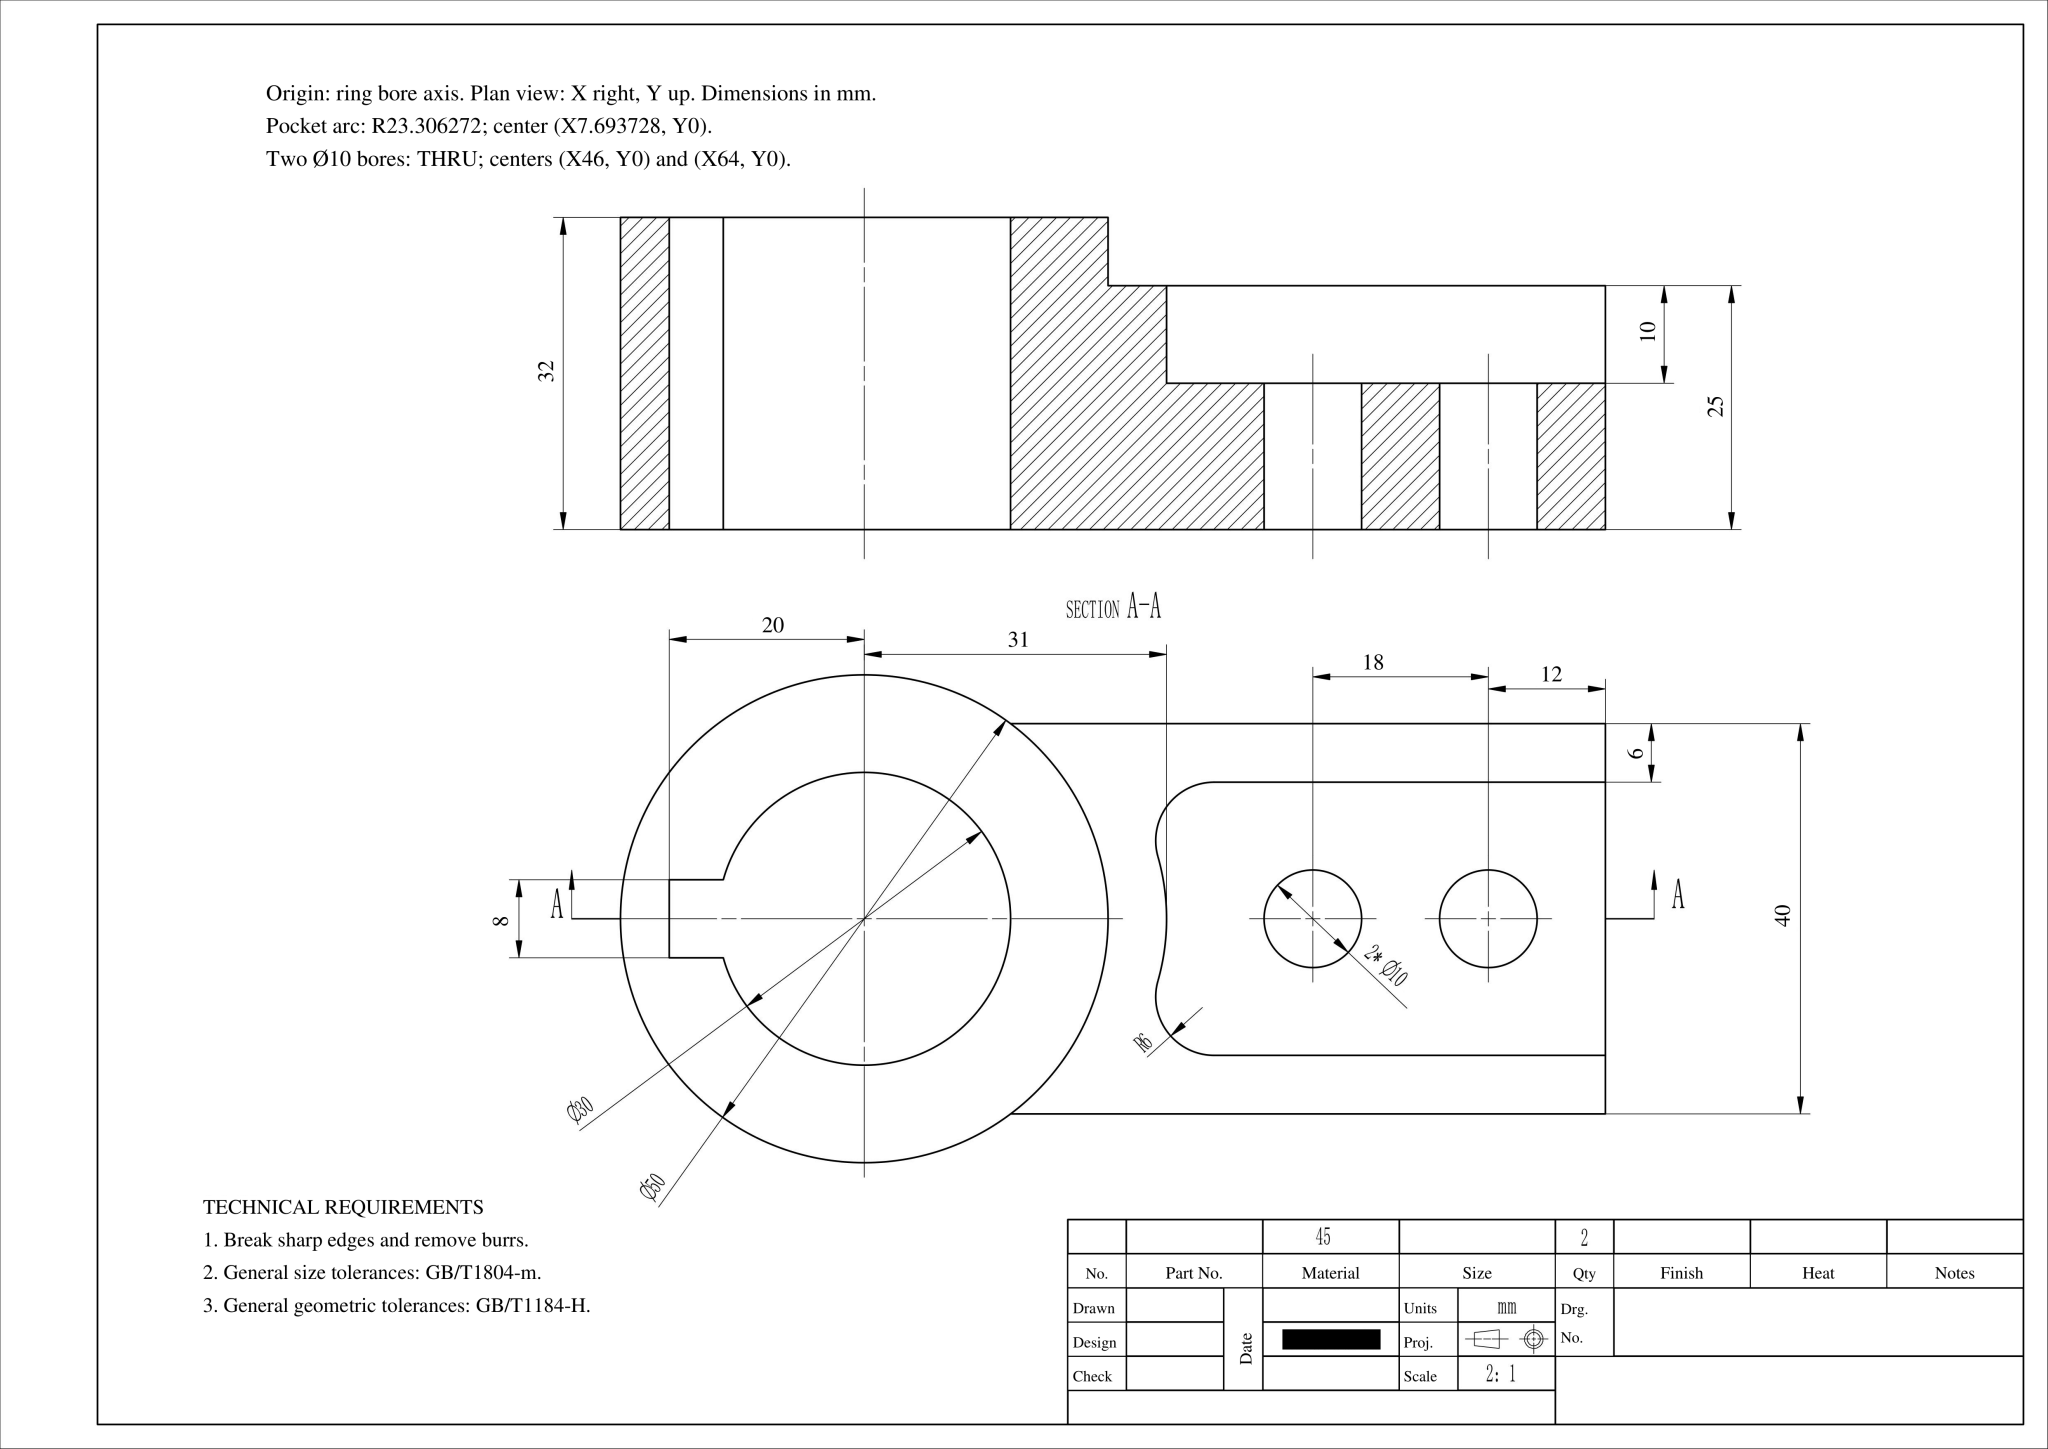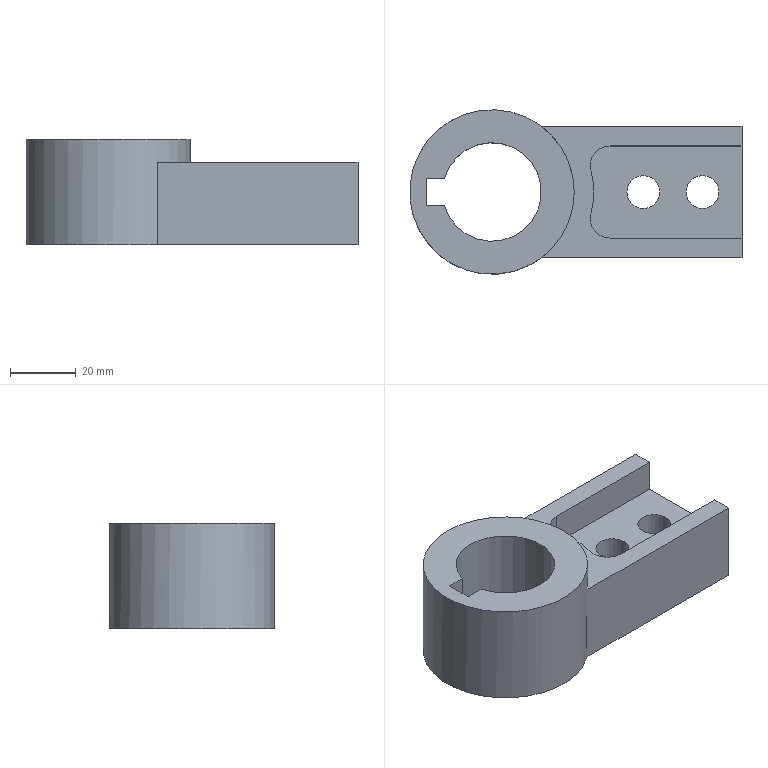Part | NX | mm | 1 solid | 19 faces | box 101 x 50 x 32 mm | volume 77891 mm3 | plane 12 | cylinder 7 | commonest cylinder face diameters 12 x2 10 x2 46.613 x1 50 x1 30 x1
STEP:
#1=CARTESIAN_POINT('',(0.,0.,0.));
#2=DIRECTION('',(0.,0.,1.));
#3=DIRECTION('',(1.,0.,0.));
#4=AXIS2_PLACEMENT_3D('',#1,#2,#3);
#5=(LENGTH_UNIT()NAMED_UNIT(*)SI_UNIT(.MILLI.,.METRE.));
#6=UNCERTAINTY_MEASURE_WITH_UNIT(LENGTH_MEASURE(0.00002),#5,'','');
#7=(NAMED_UNIT(*)PLANE_ANGLE_UNIT()SI_UNIT($,.RADIAN.));
#8=PLANE_ANGLE_MEASURE_WITH_UNIT(PLANE_ANGLE_MEASURE(0.01745),#7);
#9=DIMENSIONAL_EXPONENTS(0.,0.,0.,0.,0.,0.,0.);
#10=(CONVERSION_BASED_UNIT('',#8)NAMED_UNIT(#9)PLANE_ANGLE_UNIT());
#11=(NAMED_UNIT(*)SI_UNIT($,.STERADIAN.)SOLID_ANGLE_UNIT());
#12=(GEOMETRIC_REPRESENTATION_CONTEXT(3)GLOBAL_UNCERTAINTY_ASSIGNED_CONTEXT((#6))GLOBAL_UNIT_ASSIGNED_CONTEXT((#5,#10,#11))REPRESENTATION_CONTEXT('',''));
#13=SHAPE_REPRESENTATION('',(#4),#12);
#14=CARTESIAN_POINT('',(35.887,-14.,15.));
#15=VERTEX_POINT('',#14);
#16=CARTESIAN_POINT('',(76.,-14.,15.));
#17=VERTEX_POINT('',#16);
#18=CARTESIAN_POINT('',(35.887,-14.,15.));
#19=DIRECTION('',(1.,0.,0.));
#20=VECTOR('',#19,1.);
#21=LINE('',#18,#20);
#22=EDGE_CURVE('',#15,#17,#21,.T.);
#23=ORIENTED_EDGE('',*,*,#22,.F.);
#24=CARTESIAN_POINT('',(35.887,-14.,25.));
#25=VERTEX_POINT('',#24);
#26=CARTESIAN_POINT('',(35.887,-14.,25.));
#27=DIRECTION('',(0.,0.,-1.));
#28=VECTOR('',#27,1.);
#29=LINE('',#26,#28);
#30=EDGE_CURVE('',#25,#15,#29,.T.);
#31=ORIENTED_EDGE('',*,*,#30,.F.);
#32=CARTESIAN_POINT('',(76.,-14.,25.));
#33=VERTEX_POINT('',#32);
#34=CARTESIAN_POINT('',(76.,-14.,25.));
#35=DIRECTION('',(-1.,0.,0.));
#36=VECTOR('',#35,1.);
#37=LINE('',#34,#36);
#38=EDGE_CURVE('',#33,#25,#37,.T.);
#39=ORIENTED_EDGE('',*,*,#38,.F.);
#40=CARTESIAN_POINT('',(76.,-14.,25.));
#41=DIRECTION('',(0.,0.,-1.));
#42=VECTOR('',#41,1.);
#43=LINE('',#40,#42);
#44=EDGE_CURVE('',#33,#17,#43,.T.);
#45=ORIENTED_EDGE('',*,*,#44,.T.);
#46=EDGE_LOOP('',(#23,#31,#39,#45));
#47=FACE_OUTER_BOUND('',#46,.T.);
#48=CARTESIAN_POINT('',(76.,-14.,25.));
#49=DIRECTION('',(0.,-1.,0.));
#50=DIRECTION('',(0.,0.,-1.));
#51=AXIS2_PLACEMENT_3D('',#48,#49,#50);
#52=PLANE('',#51);
#53=ADVANCED_FACE('',(#47),#52,.F.);
#54=CARTESIAN_POINT('',(76.,14.,15.));
#55=VERTEX_POINT('',#54);
#56=CARTESIAN_POINT('',(35.887,14.,15.));
#57=VERTEX_POINT('',#56);
#58=CARTESIAN_POINT('',(76.,14.,15.));
#59=DIRECTION('',(-1.,0.,0.));
#60=VECTOR('',#59,1.);
#61=LINE('',#58,#60);
#62=EDGE_CURVE('',#55,#57,#61,.T.);
#63=ORIENTED_EDGE('',*,*,#62,.F.);
#64=CARTESIAN_POINT('',(76.,14.,25.));
#65=VERTEX_POINT('',#64);
#66=CARTESIAN_POINT('',(76.,14.,25.));
#67=DIRECTION('',(0.,0.,-1.));
#68=VECTOR('',#67,1.);
#69=LINE('',#66,#68);
#70=EDGE_CURVE('',#65,#55,#69,.T.);
#71=ORIENTED_EDGE('',*,*,#70,.F.);
#72=CARTESIAN_POINT('',(35.887,14.,25.));
#73=VERTEX_POINT('',#72);
#74=CARTESIAN_POINT('',(35.887,14.,25.));
#75=DIRECTION('',(1.,-0.,0.));
#76=VECTOR('',#75,1.);
#77=LINE('',#74,#76);
#78=EDGE_CURVE('',#73,#65,#77,.T.);
#79=ORIENTED_EDGE('',*,*,#78,.F.);
#80=CARTESIAN_POINT('',(35.887,14.,25.));
#81=DIRECTION('',(0.,0.,-1.));
#82=VECTOR('',#81,1.);
#83=LINE('',#80,#82);
#84=EDGE_CURVE('',#73,#57,#83,.T.);
#85=ORIENTED_EDGE('',*,*,#84,.T.);
#86=EDGE_LOOP('',(#63,#71,#79,#85));
#87=FACE_OUTER_BOUND('',#86,.T.);
#88=CARTESIAN_POINT('',(35.887,14.,25.));
#89=DIRECTION('',(0.,1.,0.));
#90=DIRECTION('',(-1.,0.,0.));
#91=AXIS2_PLACEMENT_3D('',#88,#89,#90);
#92=PLANE('',#91);
#93=ADVANCED_FACE('',(#87),#92,.F.);
#94=CARTESIAN_POINT('',(30.115,-6.362,15.));
#95=VERTEX_POINT('',#94);
#96=CARTESIAN_POINT('',(35.887,-8.,15.));
#97=DIRECTION('',(0.,0.,1.));
#98=DIRECTION('',(1.,0.,0.));
#99=AXIS2_PLACEMENT_3D('',#96,#97,#98);
#100=CIRCLE('',#99,6.);
#101=EDGE_CURVE('',#95,#15,#100,.T.);
#102=ORIENTED_EDGE('',*,*,#101,.F.);
#103=CARTESIAN_POINT('',(30.115,-6.362,25.));
#104=VERTEX_POINT('',#103);
#105=CARTESIAN_POINT('',(30.115,-6.362,25.));
#106=DIRECTION('',(0.,0.,-1.));
#107=VECTOR('',#106,1.);
#108=LINE('',#105,#107);
#109=EDGE_CURVE('',#104,#95,#108,.T.);
#110=ORIENTED_EDGE('',*,*,#109,.F.);
#111=CARTESIAN_POINT('',(35.887,-8.,25.));
#112=DIRECTION('',(0.,0.,-1.));
#113=DIRECTION('',(1.,0.,0.));
#114=AXIS2_PLACEMENT_3D('',#111,#112,#113);
#115=CIRCLE('',#114,6.);
#116=EDGE_CURVE('',#25,#104,#115,.T.);
#117=ORIENTED_EDGE('',*,*,#116,.F.);
#118=ORIENTED_EDGE('',*,*,#30,.T.);
#119=EDGE_LOOP('',(#102,#110,#117,#118));
#120=FACE_OUTER_BOUND('',#119,.T.);
#121=CARTESIAN_POINT('',(35.887,-8.,25.));
#122=DIRECTION('',(0.,0.,-1.));
#123=DIRECTION('',(-1.,0.,0.));
#124=AXIS2_PLACEMENT_3D('',#121,#122,#123);
#125=CYLINDRICAL_SURFACE('',#124,6.);
#126=ADVANCED_FACE('',(#120),#125,.F.);
#127=CARTESIAN_POINT('',(30.115,6.362,15.));
#128=VERTEX_POINT('',#127);
#129=CARTESIAN_POINT('',(7.694,0.,15.));
#130=DIRECTION('',(0.,0.,-1.));
#131=DIRECTION('',(1.,0.,0.));
#132=AXIS2_PLACEMENT_3D('',#129,#130,#131);
#133=CIRCLE('',#132,23.306);
#134=EDGE_CURVE('',#128,#95,#133,.T.);
#135=ORIENTED_EDGE('',*,*,#134,.F.);
#136=CARTESIAN_POINT('',(30.115,6.362,25.));
#137=VERTEX_POINT('',#136);
#138=CARTESIAN_POINT('',(30.115,6.362,25.));
#139=DIRECTION('',(0.,0.,-1.));
#140=VECTOR('',#139,1.);
#141=LINE('',#138,#140);
#142=EDGE_CURVE('',#137,#128,#141,.T.);
#143=ORIENTED_EDGE('',*,*,#142,.F.);
#144=CARTESIAN_POINT('',(7.694,0.,25.));
#145=DIRECTION('',(0.,0.,1.));
#146=DIRECTION('',(1.,0.,0.));
#147=AXIS2_PLACEMENT_3D('',#144,#145,#146);
#148=CIRCLE('',#147,23.306);
#149=EDGE_CURVE('',#104,#137,#148,.T.);
#150=ORIENTED_EDGE('',*,*,#149,.F.);
#151=ORIENTED_EDGE('',*,*,#109,.T.);
#152=EDGE_LOOP('',(#135,#143,#150,#151));
#153=FACE_OUTER_BOUND('',#152,.T.);
#154=CARTESIAN_POINT('',(7.694,0.,25.));
#155=DIRECTION('',(0.,0.,-1.));
#156=DIRECTION('',(-1.,0.,0.));
#157=AXIS2_PLACEMENT_3D('',#154,#155,#156);
#158=CYLINDRICAL_SURFACE('',#157,23.306);
#159=ADVANCED_FACE('',(#153),#158,.T.);
#160=CARTESIAN_POINT('',(35.887,8.,15.));
#161=DIRECTION('',(0.,0.,1.));
#162=DIRECTION('',(1.,0.,0.));
#163=AXIS2_PLACEMENT_3D('',#160,#161,#162);
#164=CIRCLE('',#163,6.);
#165=EDGE_CURVE('',#57,#128,#164,.T.);
#166=ORIENTED_EDGE('',*,*,#165,.F.);
#167=ORIENTED_EDGE('',*,*,#84,.F.);
#168=CARTESIAN_POINT('',(35.887,8.,25.));
#169=DIRECTION('',(0.,0.,-1.));
#170=DIRECTION('',(1.,0.,0.));
#171=AXIS2_PLACEMENT_3D('',#168,#169,#170);
#172=CIRCLE('',#171,6.);
#173=EDGE_CURVE('',#137,#73,#172,.T.);
#174=ORIENTED_EDGE('',*,*,#173,.F.);
#175=ORIENTED_EDGE('',*,*,#142,.T.);
#176=EDGE_LOOP('',(#166,#167,#174,#175));
#177=FACE_OUTER_BOUND('',#176,.T.);
#178=CARTESIAN_POINT('',(35.887,8.,25.));
#179=DIRECTION('',(0.,0.,-1.));
#180=DIRECTION('',(-1.,0.,0.));
#181=AXIS2_PLACEMENT_3D('',#178,#179,#180);
#182=CYLINDRICAL_SURFACE('',#181,6.);
#183=ADVANCED_FACE('',(#177),#182,.F.);
#184=CARTESIAN_POINT('',(25.,0.,32.));
#185=VERTEX_POINT('',#184);
#186=CARTESIAN_POINT('',(0.,0.,32.));
#187=DIRECTION('',(0.,0.,1.));
#188=DIRECTION('',(1.,0.,0.));
#189=AXIS2_PLACEMENT_3D('',#186,#187,#188);
#190=CIRCLE('',#189,25.);
#191=EDGE_CURVE('',#185,#185,#190,.T.);
#192=ORIENTED_EDGE('',*,*,#191,.F.);
#193=EDGE_LOOP('',(#192));
#194=FACE_BOUND('',#193,.T.);
#195=CARTESIAN_POINT('',(15.,-20.,25.));
#196=VERTEX_POINT('',#195);
#197=CARTESIAN_POINT('',(15.,-20.,0.));
#198=VERTEX_POINT('',#197);
#199=CARTESIAN_POINT('',(15.,-20.,25.));
#200=DIRECTION('',(0.,0.,-1.));
#201=VECTOR('',#200,1.);
#202=LINE('',#199,#201);
#203=EDGE_CURVE('',#196,#198,#202,.T.);
#204=ORIENTED_EDGE('',*,*,#203,.F.);
#205=CARTESIAN_POINT('',(15.,20.,25.));
#206=VERTEX_POINT('',#205);
#207=CARTESIAN_POINT('',(0.,0.,25.));
#208=DIRECTION('',(0.,0.,-1.));
#209=DIRECTION('',(1.,0.,0.));
#210=AXIS2_PLACEMENT_3D('',#207,#208,#209);
#211=CIRCLE('',#210,25.);
#212=EDGE_CURVE('',#206,#196,#211,.T.);
#213=ORIENTED_EDGE('',*,*,#212,.F.);
#214=CARTESIAN_POINT('',(15.,20.,0.));
#215=VERTEX_POINT('',#214);
#216=CARTESIAN_POINT('',(15.,20.,25.));
#217=DIRECTION('',(0.,0.,-1.));
#218=VECTOR('',#217,1.);
#219=LINE('',#216,#218);
#220=EDGE_CURVE('',#206,#215,#219,.T.);
#221=ORIENTED_EDGE('',*,*,#220,.T.);
#222=CARTESIAN_POINT('',(0.,0.,0.));
#223=DIRECTION('',(0.,0.,1.));
#224=DIRECTION('',(1.,0.,0.));
#225=AXIS2_PLACEMENT_3D('',#222,#223,#224);
#226=CIRCLE('',#225,25.);
#227=EDGE_CURVE('',#215,#198,#226,.T.);
#228=ORIENTED_EDGE('',*,*,#227,.T.);
#229=EDGE_LOOP('',(#204,#213,#221,#228));
#230=FACE_BOUND('',#229,.T.);
#231=CARTESIAN_POINT('',(0.,0.,32.));
#232=DIRECTION('',(0.,0.,-1.));
#233=DIRECTION('',(-1.,0.,0.));
#234=AXIS2_PLACEMENT_3D('',#231,#232,#233);
#235=CYLINDRICAL_SURFACE('',#234,25.);
#236=ADVANCED_FACE('',(#194,#230),#235,.T.);
#237=CARTESIAN_POINT('',(-20.,-4.,0.));
#238=VERTEX_POINT('',#237);
#239=CARTESIAN_POINT('',(-20.,4.,0.));
#240=VERTEX_POINT('',#239);
#241=CARTESIAN_POINT('',(-20.,-4.,0.));
#242=DIRECTION('',(0.,1.,0.));
#243=VECTOR('',#242,1.);
#244=LINE('',#241,#243);
#245=EDGE_CURVE('',#238,#240,#244,.T.);
#246=ORIENTED_EDGE('',*,*,#245,.T.);
#247=CARTESIAN_POINT('',(-20.,4.,32.));
#248=VERTEX_POINT('',#247);
#249=CARTESIAN_POINT('',(-20.,4.,32.));
#250=DIRECTION('',(0.,0.,-1.));
#251=VECTOR('',#250,1.);
#252=LINE('',#249,#251);
#253=EDGE_CURVE('',#248,#240,#252,.T.);
#254=ORIENTED_EDGE('',*,*,#253,.F.);
#255=CARTESIAN_POINT('',(-20.,-4.,32.));
#256=VERTEX_POINT('',#255);
#257=CARTESIAN_POINT('',(-20.,-4.,32.));
#258=DIRECTION('',(0.,1.,0.));
#259=VECTOR('',#258,1.);
#260=LINE('',#257,#259);
#261=EDGE_CURVE('',#256,#248,#260,.T.);
#262=ORIENTED_EDGE('',*,*,#261,.F.);
#263=CARTESIAN_POINT('',(-20.,-4.,32.));
#264=DIRECTION('',(0.,0.,-1.));
#265=VECTOR('',#264,1.);
#266=LINE('',#263,#265);
#267=EDGE_CURVE('',#256,#238,#266,.T.);
#268=ORIENTED_EDGE('',*,*,#267,.T.);
#269=EDGE_LOOP('',(#246,#254,#262,#268));
#270=FACE_OUTER_BOUND('',#269,.T.);
#271=CARTESIAN_POINT('',(-20.,-4.,32.));
#272=DIRECTION('',(-1.,0.,0.));
#273=DIRECTION('',(-0.,-1.,0.));
#274=AXIS2_PLACEMENT_3D('',#271,#272,#273);
#275=PLANE('',#274);
#276=ADVANCED_FACE('',(#270),#275,.F.);
#277=CARTESIAN_POINT('',(-14.457,4.,0.));
#278=VERTEX_POINT('',#277);
#279=CARTESIAN_POINT('',(-20.,4.,0.));
#280=DIRECTION('',(1.,0.,0.));
#281=VECTOR('',#280,1.);
#282=LINE('',#279,#281);
#283=EDGE_CURVE('',#240,#278,#282,.T.);
#284=ORIENTED_EDGE('',*,*,#283,.T.);
#285=CARTESIAN_POINT('',(-14.457,4.,32.));
#286=VERTEX_POINT('',#285);
#287=CARTESIAN_POINT('',(-14.457,4.,32.));
#288=DIRECTION('',(0.,0.,-1.));
#289=VECTOR('',#288,1.);
#290=LINE('',#287,#289);
#291=EDGE_CURVE('',#286,#278,#290,.T.);
#292=ORIENTED_EDGE('',*,*,#291,.F.);
#293=CARTESIAN_POINT('',(-20.,4.,32.));
#294=DIRECTION('',(1.,0.,0.));
#295=VECTOR('',#294,1.);
#296=LINE('',#293,#295);
#297=EDGE_CURVE('',#248,#286,#296,.T.);
#298=ORIENTED_EDGE('',*,*,#297,.F.);
#299=ORIENTED_EDGE('',*,*,#253,.T.);
#300=EDGE_LOOP('',(#284,#292,#298,#299));
#301=FACE_OUTER_BOUND('',#300,.T.);
#302=CARTESIAN_POINT('',(-20.,4.,32.));
#303=DIRECTION('',(0.,1.,0.));
#304=DIRECTION('',(0.,0.,1.));
#305=AXIS2_PLACEMENT_3D('',#302,#303,#304);
#306=PLANE('',#305);
#307=ADVANCED_FACE('',(#301),#306,.F.);
#308=CARTESIAN_POINT('',(-14.457,-4.,0.));
#309=VERTEX_POINT('',#308);
#310=CARTESIAN_POINT('',(0.,0.,0.));
#311=DIRECTION('',(0.,0.,-1.));
#312=DIRECTION('',(1.,0.,0.));
#313=AXIS2_PLACEMENT_3D('',#310,#311,#312);
#314=CIRCLE('',#313,15.);
#315=EDGE_CURVE('',#278,#309,#314,.T.);
#316=ORIENTED_EDGE('',*,*,#315,.T.);
#317=CARTESIAN_POINT('',(-14.457,-4.,32.));
#318=VERTEX_POINT('',#317);
#319=CARTESIAN_POINT('',(-14.457,-4.,32.));
#320=DIRECTION('',(0.,0.,-1.));
#321=VECTOR('',#320,1.);
#322=LINE('',#319,#321);
#323=EDGE_CURVE('',#318,#309,#322,.T.);
#324=ORIENTED_EDGE('',*,*,#323,.F.);
#325=CARTESIAN_POINT('',(0.,0.,32.));
#326=DIRECTION('',(0.,0.,-1.));
#327=DIRECTION('',(1.,0.,0.));
#328=AXIS2_PLACEMENT_3D('',#325,#326,#327);
#329=CIRCLE('',#328,15.);
#330=EDGE_CURVE('',#286,#318,#329,.T.);
#331=ORIENTED_EDGE('',*,*,#330,.F.);
#332=ORIENTED_EDGE('',*,*,#291,.T.);
#333=EDGE_LOOP('',(#316,#324,#331,#332));
#334=FACE_OUTER_BOUND('',#333,.T.);
#335=CARTESIAN_POINT('',(0.,0.,32.));
#336=DIRECTION('',(0.,0.,-1.));
#337=DIRECTION('',(-1.,0.,0.));
#338=AXIS2_PLACEMENT_3D('',#335,#336,#337);
#339=CYLINDRICAL_SURFACE('',#338,15.);
#340=ADVANCED_FACE('',(#334),#339,.F.);
#341=CARTESIAN_POINT('',(-14.457,-4.,0.));
#342=DIRECTION('',(-1.,0.,0.));
#343=VECTOR('',#342,1.);
#344=LINE('',#341,#343);
#345=EDGE_CURVE('',#309,#238,#344,.T.);
#346=ORIENTED_EDGE('',*,*,#345,.T.);
#347=ORIENTED_EDGE('',*,*,#267,.F.);
#348=CARTESIAN_POINT('',(-14.457,-4.,32.));
#349=DIRECTION('',(-1.,0.,0.));
#350=VECTOR('',#349,1.);
#351=LINE('',#348,#350);
#352=EDGE_CURVE('',#318,#256,#351,.T.);
#353=ORIENTED_EDGE('',*,*,#352,.F.);
#354=ORIENTED_EDGE('',*,*,#323,.T.);
#355=EDGE_LOOP('',(#346,#347,#353,#354));
#356=FACE_OUTER_BOUND('',#355,.T.);
#357=CARTESIAN_POINT('',(-14.457,-4.,32.));
#358=DIRECTION('',(0.,-1.,0.));
#359=DIRECTION('',(0.,0.,-1.));
#360=AXIS2_PLACEMENT_3D('',#357,#358,#359);
#361=PLANE('',#360);
#362=ADVANCED_FACE('',(#356),#361,.F.);
#363=ORIENTED_EDGE('',*,*,#191,.T.);
#364=EDGE_LOOP('',(#363));
#365=FACE_BOUND('',#364,.T.);
#366=ORIENTED_EDGE('',*,*,#261,.T.);
#367=ORIENTED_EDGE('',*,*,#297,.T.);
#368=ORIENTED_EDGE('',*,*,#330,.T.);
#369=ORIENTED_EDGE('',*,*,#352,.T.);
#370=EDGE_LOOP('',(#366,#367,#368,#369));
#371=FACE_BOUND('',#370,.T.);
#372=CARTESIAN_POINT('',(0.,0.,32.));
#373=DIRECTION('',(0.,0.,1.));
#374=DIRECTION('',(1.,0.,0.));
#375=AXIS2_PLACEMENT_3D('',#372,#373,#374);
#376=PLANE('',#375);
#377=ADVANCED_FACE('',(#365,#371),#376,.T.);
#378=CARTESIAN_POINT('',(76.,20.,0.));
#379=VERTEX_POINT('',#378);
#380=CARTESIAN_POINT('',(76.,20.,0.));
#381=DIRECTION('',(-1.,0.,0.));
#382=VECTOR('',#381,1.);
#383=LINE('',#380,#382);
#384=EDGE_CURVE('',#379,#215,#383,.T.);
#385=ORIENTED_EDGE('',*,*,#384,.F.);
#386=CARTESIAN_POINT('',(76.,-20.,0.));
#387=VERTEX_POINT('',#386);
#388=CARTESIAN_POINT('',(76.,-20.,0.));
#389=DIRECTION('',(0.,1.,0.));
#390=VECTOR('',#389,1.);
#391=LINE('',#388,#390);
#392=EDGE_CURVE('',#387,#379,#391,.T.);
#393=ORIENTED_EDGE('',*,*,#392,.F.);
#394=CARTESIAN_POINT('',(15.,-20.,0.));
#395=DIRECTION('',(1.,0.,0.));
#396=VECTOR('',#395,1.);
#397=LINE('',#394,#396);
#398=EDGE_CURVE('',#198,#387,#397,.T.);
#399=ORIENTED_EDGE('',*,*,#398,.F.);
#400=ORIENTED_EDGE('',*,*,#227,.F.);
#401=EDGE_LOOP('',(#385,#393,#399,#400));
#402=FACE_BOUND('',#401,.T.);
#403=ORIENTED_EDGE('',*,*,#245,.F.);
#404=ORIENTED_EDGE('',*,*,#345,.F.);
#405=ORIENTED_EDGE('',*,*,#315,.F.);
#406=ORIENTED_EDGE('',*,*,#283,.F.);
#407=EDGE_LOOP('',(#403,#404,#405,#406));
#408=FACE_BOUND('',#407,.T.);
#409=CARTESIAN_POINT('',(51.,0.,0.));
#410=VERTEX_POINT('',#409);
#411=CARTESIAN_POINT('',(46.,0.,0.));
#412=DIRECTION('',(0.,0.,1.));
#413=DIRECTION('',(1.,0.,0.));
#414=AXIS2_PLACEMENT_3D('',#411,#412,#413);
#415=CIRCLE('',#414,5.);
#416=EDGE_CURVE('',#410,#410,#415,.T.);
#417=ORIENTED_EDGE('',*,*,#416,.T.);
#418=EDGE_LOOP('',(#417));
#419=FACE_BOUND('',#418,.T.);
#420=CARTESIAN_POINT('',(69.,0.,0.));
#421=VERTEX_POINT('',#420);
#422=CARTESIAN_POINT('',(64.,0.,0.));
#423=DIRECTION('',(0.,0.,1.));
#424=DIRECTION('',(1.,0.,0.));
#425=AXIS2_PLACEMENT_3D('',#422,#423,#424);
#426=CIRCLE('',#425,5.);
#427=EDGE_CURVE('',#421,#421,#426,.T.);
#428=ORIENTED_EDGE('',*,*,#427,.T.);
#429=EDGE_LOOP('',(#428));
#430=FACE_BOUND('',#429,.T.);
#431=CARTESIAN_POINT('',(0.,0.,0.));
#432=DIRECTION('',(0.,0.,1.));
#433=DIRECTION('',(1.,0.,0.));
#434=AXIS2_PLACEMENT_3D('',#431,#432,#433);
#435=PLANE('',#434);
#436=ADVANCED_FACE('',(#402,#408,#419,#430),#435,.F.);
#437=ORIENTED_EDGE('',*,*,#398,.T.);
#438=CARTESIAN_POINT('',(76.,-20.,25.));
#439=VERTEX_POINT('',#438);
#440=CARTESIAN_POINT('',(76.,-20.,25.));
#441=DIRECTION('',(0.,0.,-1.));
#442=VECTOR('',#441,1.);
#443=LINE('',#440,#442);
#444=EDGE_CURVE('',#439,#387,#443,.T.);
#445=ORIENTED_EDGE('',*,*,#444,.F.);
#446=CARTESIAN_POINT('',(15.,-20.,25.));
#447=DIRECTION('',(1.,0.,0.));
#448=VECTOR('',#447,1.);
#449=LINE('',#446,#448);
#450=EDGE_CURVE('',#196,#439,#449,.T.);
#451=ORIENTED_EDGE('',*,*,#450,.F.);
#452=ORIENTED_EDGE('',*,*,#203,.T.);
#453=EDGE_LOOP('',(#437,#445,#451,#452));
#454=FACE_OUTER_BOUND('',#453,.T.);
#455=CARTESIAN_POINT('',(15.,-20.,25.));
#456=DIRECTION('',(-0.,1.,0.));
#457=DIRECTION('',(-1.,-0.,0.));
#458=AXIS2_PLACEMENT_3D('',#455,#456,#457);
#459=PLANE('',#458);
#460=ADVANCED_FACE('',(#454),#459,.F.);
#461=ORIENTED_EDGE('',*,*,#392,.T.);
#462=CARTESIAN_POINT('',(76.,20.,25.));
#463=VERTEX_POINT('',#462);
#464=CARTESIAN_POINT('',(76.,20.,25.));
#465=DIRECTION('',(0.,0.,-1.));
#466=VECTOR('',#465,1.);
#467=LINE('',#464,#466);
#468=EDGE_CURVE('',#463,#379,#467,.T.);
#469=ORIENTED_EDGE('',*,*,#468,.F.);
#470=CARTESIAN_POINT('',(76.,14.,25.));
#471=DIRECTION('',(0.,1.,0.));
#472=VECTOR('',#471,1.);
#473=LINE('',#470,#472);
#474=EDGE_CURVE('',#65,#463,#473,.T.);
#475=ORIENTED_EDGE('',*,*,#474,.F.);
#476=ORIENTED_EDGE('',*,*,#70,.T.);
#477=CARTESIAN_POINT('',(76.,-14.,15.));
#478=DIRECTION('',(0.,1.,0.));
#479=VECTOR('',#478,1.);
#480=LINE('',#477,#479);
#481=EDGE_CURVE('',#17,#55,#480,.T.);
#482=ORIENTED_EDGE('',*,*,#481,.F.);
#483=ORIENTED_EDGE('',*,*,#44,.F.);
#484=CARTESIAN_POINT('',(76.,-20.,25.));
#485=DIRECTION('',(0.,1.,0.));
#486=VECTOR('',#485,1.);
#487=LINE('',#484,#486);
#488=EDGE_CURVE('',#439,#33,#487,.T.);
#489=ORIENTED_EDGE('',*,*,#488,.F.);
#490=ORIENTED_EDGE('',*,*,#444,.T.);
#491=EDGE_LOOP('',(#461,#469,#475,#476,#482,#483,#489,#490));
#492=FACE_OUTER_BOUND('',#491,.T.);
#493=CARTESIAN_POINT('',(76.,-20.,25.));
#494=DIRECTION('',(-1.,0.,0.));
#495=DIRECTION('',(0.,0.,1.));
#496=AXIS2_PLACEMENT_3D('',#493,#494,#495);
#497=PLANE('',#496);
#498=ADVANCED_FACE('',(#492),#497,.F.);
#499=ORIENTED_EDGE('',*,*,#384,.T.);
#500=ORIENTED_EDGE('',*,*,#220,.F.);
#501=CARTESIAN_POINT('',(76.,20.,25.));
#502=DIRECTION('',(-1.,0.,0.));
#503=VECTOR('',#502,1.);
#504=LINE('',#501,#503);
#505=EDGE_CURVE('',#463,#206,#504,.T.);
#506=ORIENTED_EDGE('',*,*,#505,.F.);
#507=ORIENTED_EDGE('',*,*,#468,.T.);
#508=EDGE_LOOP('',(#499,#500,#506,#507));
#509=FACE_OUTER_BOUND('',#508,.T.);
#510=CARTESIAN_POINT('',(76.,20.,25.));
#511=DIRECTION('',(-0.,-1.,0.));
#512=DIRECTION('',(1.,-0.,0.));
#513=AXIS2_PLACEMENT_3D('',#510,#511,#512);
#514=PLANE('',#513);
#515=ADVANCED_FACE('',(#509),#514,.F.);
#516=ORIENTED_EDGE('',*,*,#212,.T.);
#517=ORIENTED_EDGE('',*,*,#450,.T.);
#518=ORIENTED_EDGE('',*,*,#488,.T.);
#519=ORIENTED_EDGE('',*,*,#38,.T.);
#520=ORIENTED_EDGE('',*,*,#116,.T.);
#521=ORIENTED_EDGE('',*,*,#149,.T.);
#522=ORIENTED_EDGE('',*,*,#173,.T.);
#523=ORIENTED_EDGE('',*,*,#78,.T.);
#524=ORIENTED_EDGE('',*,*,#474,.T.);
#525=ORIENTED_EDGE('',*,*,#505,.T.);
#526=EDGE_LOOP('',(#516,#517,#518,#519,#520,#521,#522,#523,#524,#525));
#527=FACE_OUTER_BOUND('',#526,.T.);
#528=CARTESIAN_POINT('',(0.,0.,25.));
#529=DIRECTION('',(0.,0.,-1.));
#530=DIRECTION('',(-1.,0.,0.));
#531=AXIS2_PLACEMENT_3D('',#528,#529,#530);
#532=PLANE('',#531);
#533=ADVANCED_FACE('',(#527),#532,.F.);
#534=CARTESIAN_POINT('',(51.,0.,15.));
#535=VERTEX_POINT('',#534);
#536=CARTESIAN_POINT('',(46.,0.,15.));
#537=DIRECTION('',(0.,0.,1.));
#538=DIRECTION('',(1.,0.,0.));
#539=AXIS2_PLACEMENT_3D('',#536,#537,#538);
#540=CIRCLE('',#539,5.);
#541=EDGE_CURVE('',#535,#535,#540,.T.);
#542=ORIENTED_EDGE('',*,*,#541,.T.);
#543=EDGE_LOOP('',(#542));
#544=FACE_BOUND('',#543,.T.);
#545=ORIENTED_EDGE('',*,*,#416,.F.);
#546=EDGE_LOOP('',(#545));
#547=FACE_BOUND('',#546,.T.);
#548=CARTESIAN_POINT('',(46.,0.,15.));
#549=DIRECTION('',(0.,0.,-1.));
#550=DIRECTION('',(-1.,0.,0.));
#551=AXIS2_PLACEMENT_3D('',#548,#549,#550);
#552=CYLINDRICAL_SURFACE('',#551,5.);
#553=ADVANCED_FACE('',(#544,#547),#552,.F.);
#554=CARTESIAN_POINT('',(69.,0.,15.));
#555=VERTEX_POINT('',#554);
#556=CARTESIAN_POINT('',(64.,0.,15.));
#557=DIRECTION('',(0.,0.,1.));
#558=DIRECTION('',(1.,0.,0.));
#559=AXIS2_PLACEMENT_3D('',#556,#557,#558);
#560=CIRCLE('',#559,5.);
#561=EDGE_CURVE('',#555,#555,#560,.T.);
#562=ORIENTED_EDGE('',*,*,#561,.T.);
#563=EDGE_LOOP('',(#562));
#564=FACE_BOUND('',#563,.T.);
#565=ORIENTED_EDGE('',*,*,#427,.F.);
#566=EDGE_LOOP('',(#565));
#567=FACE_BOUND('',#566,.T.);
#568=CARTESIAN_POINT('',(64.,0.,15.));
#569=DIRECTION('',(0.,0.,-1.));
#570=DIRECTION('',(-1.,0.,0.));
#571=AXIS2_PLACEMENT_3D('',#568,#569,#570);
#572=CYLINDRICAL_SURFACE('',#571,5.);
#573=ADVANCED_FACE('',(#564,#567),#572,.F.);
#574=ORIENTED_EDGE('',*,*,#134,.T.);
#575=ORIENTED_EDGE('',*,*,#101,.T.);
#576=ORIENTED_EDGE('',*,*,#22,.T.);
#577=ORIENTED_EDGE('',*,*,#481,.T.);
#578=ORIENTED_EDGE('',*,*,#62,.T.);
#579=ORIENTED_EDGE('',*,*,#165,.T.);
#580=EDGE_LOOP('',(#574,#575,#576,#577,#578,#579));
#581=FACE_BOUND('',#580,.T.);
#582=ORIENTED_EDGE('',*,*,#541,.F.);
#583=EDGE_LOOP('',(#582));
#584=FACE_BOUND('',#583,.T.);
#585=ORIENTED_EDGE('',*,*,#561,.F.);
#586=EDGE_LOOP('',(#585));
#587=FACE_BOUND('',#586,.T.);
#588=CARTESIAN_POINT('',(7.694,0.,15.));
#589=DIRECTION('',(0.,0.,-1.));
#590=DIRECTION('',(-1.,0.,0.));
#591=AXIS2_PLACEMENT_3D('',#588,#589,#590);
#592=PLANE('',#591);
#593=ADVANCED_FACE('',(#581,#584,#587),#592,.F.);
#594=CLOSED_SHELL('',(#53,#93,#126,#159,#183,#236,#276,#307,#340,#362,#377,#436,#460,#498,#515,#533,#553,#573,#593));
#595=MANIFOLD_SOLID_BREP('',#594);
#596=ADVANCED_BREP_SHAPE_REPRESENTATION('',(#595),#12);
#597=SHAPE_REPRESENTATION_RELATIONSHIP('','',#13,#596);
#598=PRESENTATION_LAYER_ASSIGNMENT('','',(#595));
#599=COLOUR_RGB('',1.,0.6,0.);
#600=FILL_AREA_STYLE_COLOUR('',#599);
#601=FILL_AREA_STYLE('',(#600));
#602=SURFACE_STYLE_FILL_AREA(#601);
#603=SURFACE_SIDE_STYLE('',(#602));
#604=SURFACE_STYLE_USAGE(.BOTH.,#603);
#605=PRESENTATION_STYLE_ASSIGNMENT((#604));
#606=STYLED_ITEM('',(#605),#595);
#607=MECHANICAL_DESIGN_GEOMETRIC_PRESENTATION_REPRESENTATION('',(#606),#12);